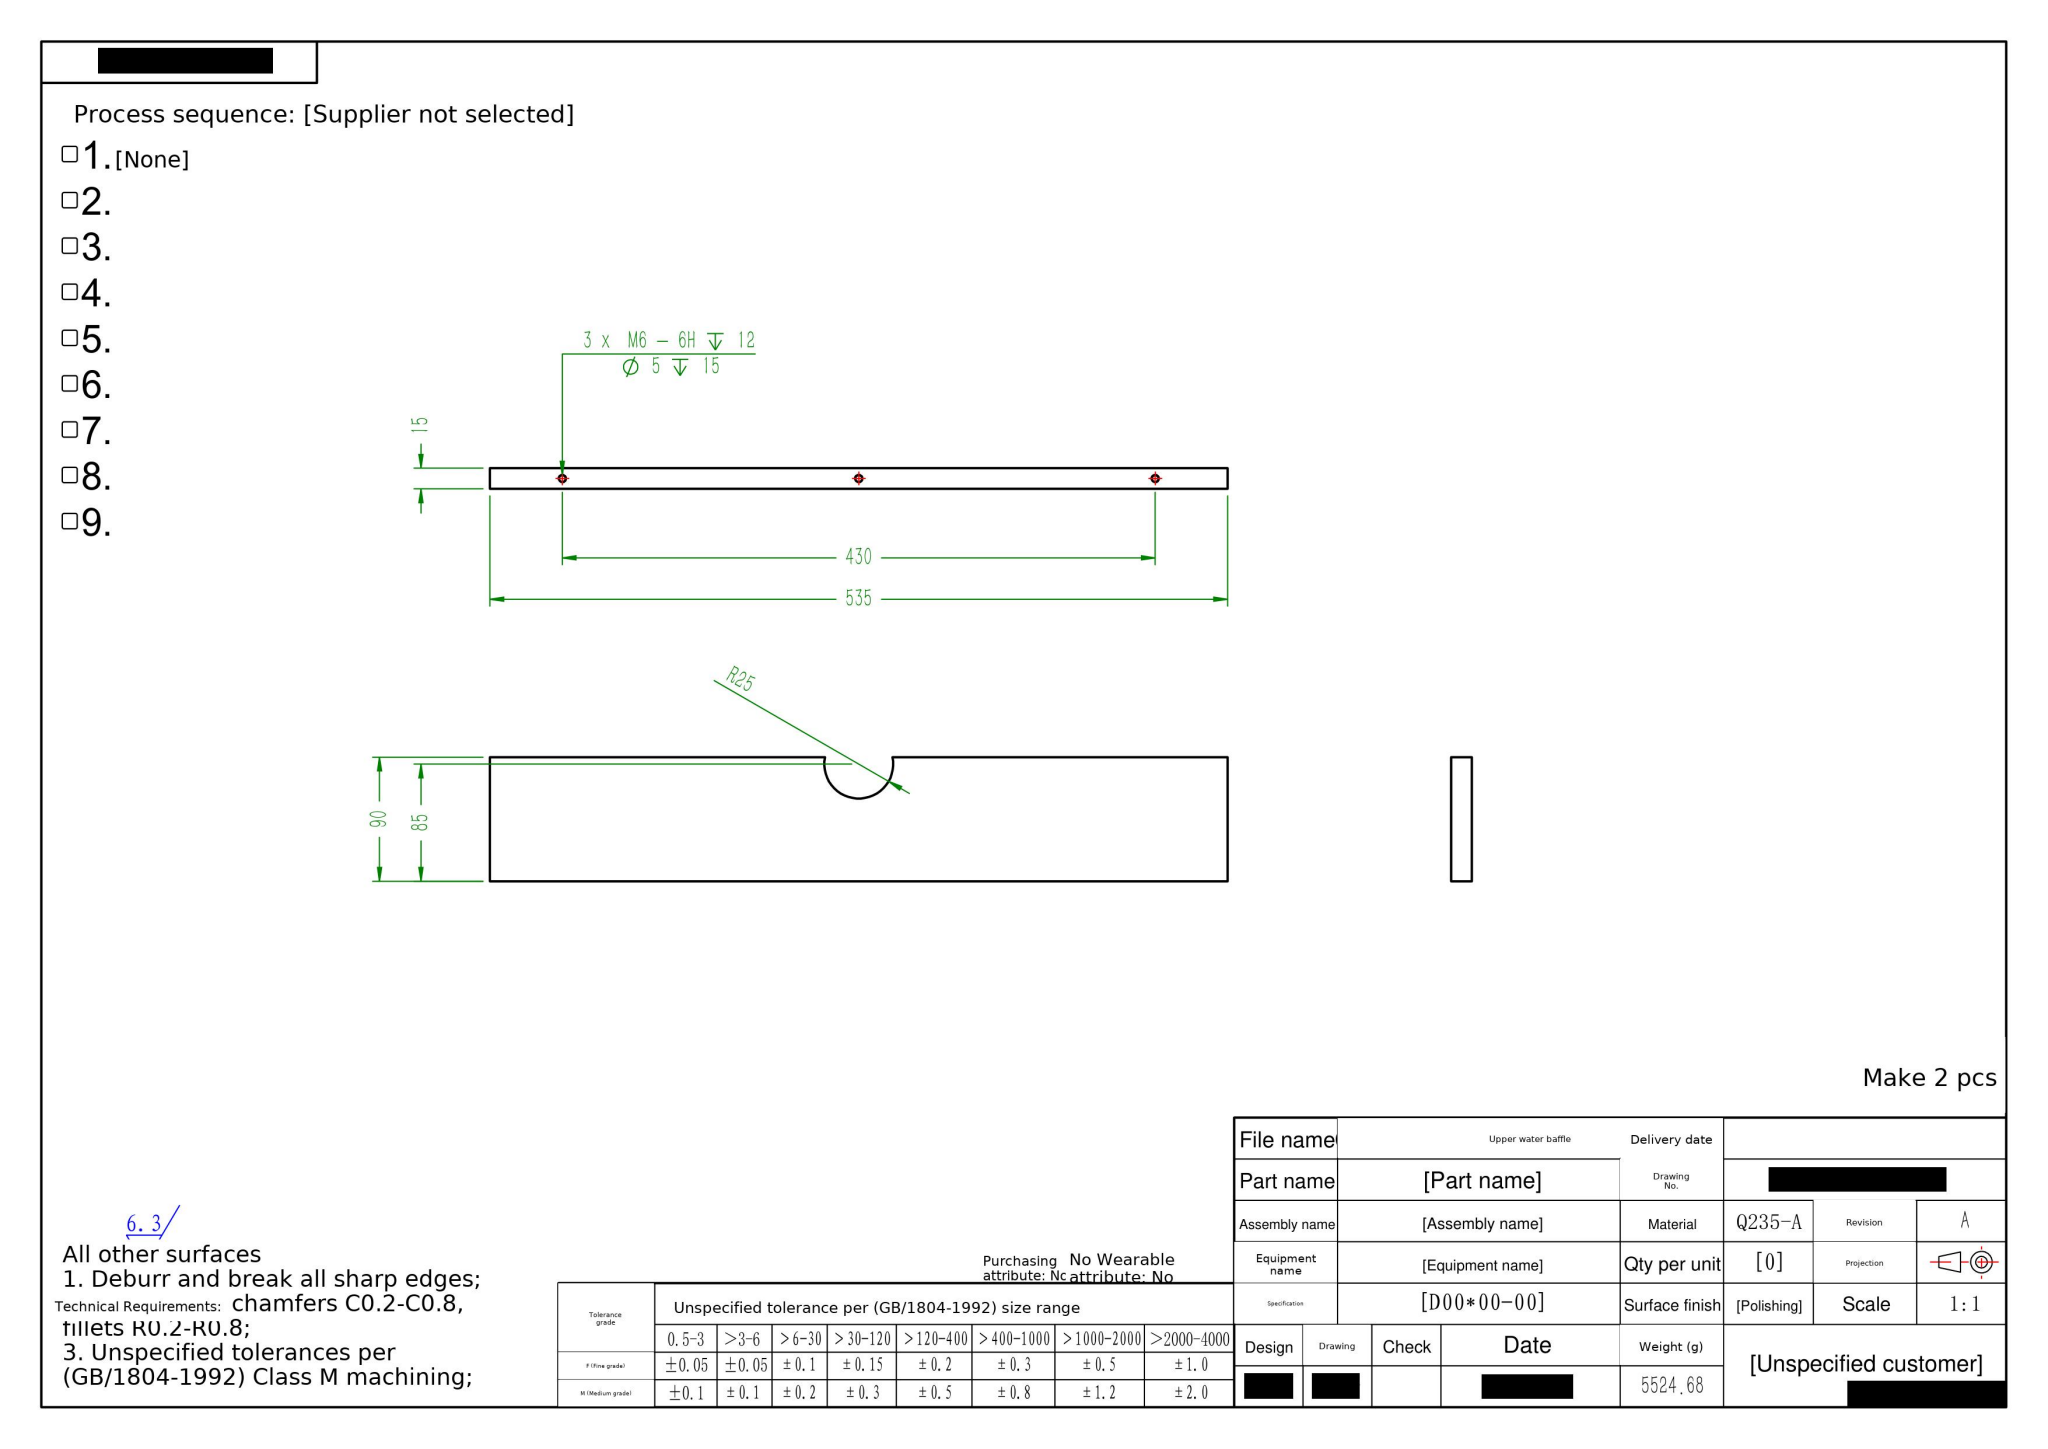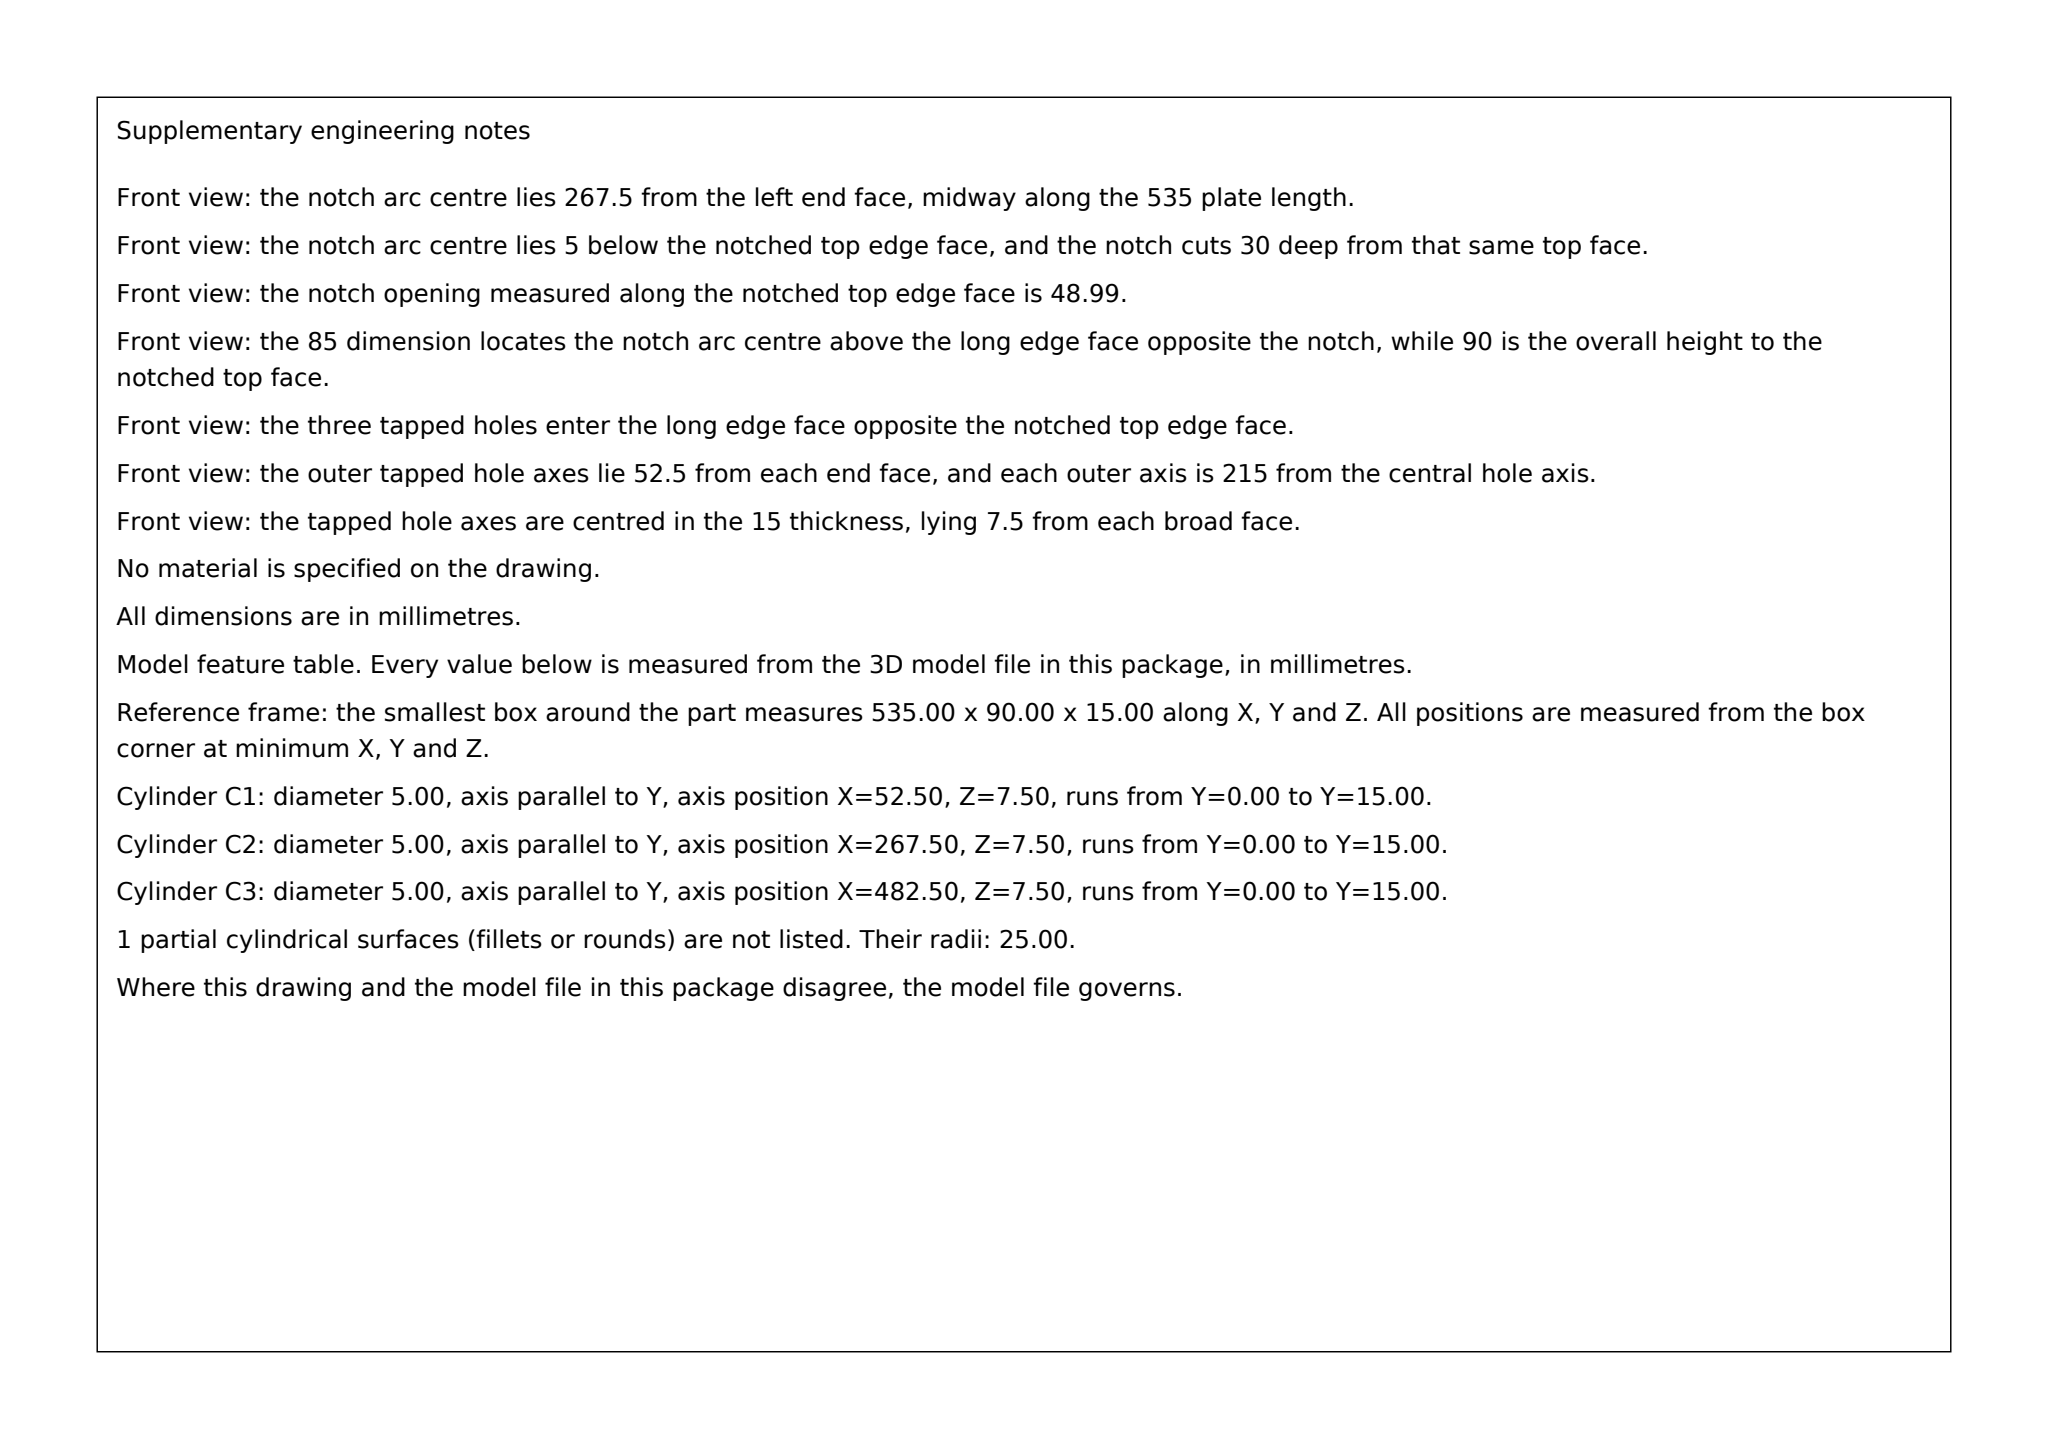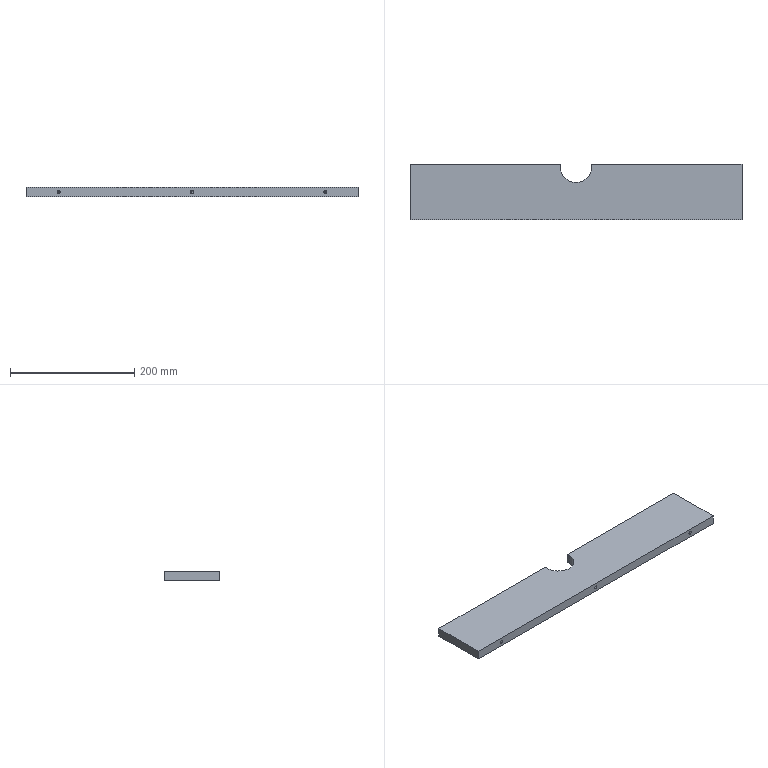Part | SolidWorks | mm | material Q235-A | 1 solid | 22 faces | box 535 x 90 x 15 mm | volume 702886 mm3 | cylinder 9 | plane 7 | cone 6 | commonest cylinder face diameters 5 x6 50 x3
Drawing notes:
2. BREAK SHARP EDGES: CHAMFERS C0.2-C0.8, FILLETS R0.2-R0.8 | from the solid: STEP lists no fillet radii (fillet_radii: []) and no chamfer faces; only sharp-edge prismatic bbox 535x90x15, so note is a general edge-break requirement
build123d program:
from build123d import *

# Parameters (mm, degrees)
SKETCH1_W             = 535
SKETCH1_H             = 15
BOSS_EXTRUDE1_DEPTH   = 90
M6_TAPPED_HOLE1_D     = 5
M6_TAPPED_HOLE1_DEPTH = 15
M6_TAPPED_HOLE1_TIP   = 1.502
SKETCH5_R             = 25
CUT_EXTRUDE2_DEPTH    = 283.633


with BuildPart() as part:
    # Sketch1 → Boss-Extrude1 (new body)
    with BuildSketch(Plane(origin=(0, 0, 0), x_dir=(1, 0, 0), z_dir=(0, 1, 0))):
        Rectangle(SKETCH1_W, SKETCH1_H)
    extrude(amount=BOSS_EXTRUDE1_DEPTH)

    # M6 Tapped Hole1
    with Locations(Plane(origin=(0, 0, 0), x_dir=(-1, 0, 0), z_dir=(0, -1, 0))):
        with Locations((0, 0), (-215, 0), (215, 0)):
            Hole(M6_TAPPED_HOLE1_D / 2, depth=M6_TAPPED_HOLE1_DEPTH)
            with Locations((0, 0, -(M6_TAPPED_HOLE1_DEPTH + M6_TAPPED_HOLE1_TIP / 2))):  # 118° drill point
                Cone(0, M6_TAPPED_HOLE1_D / 2, M6_TAPPED_HOLE1_TIP, mode=Mode.SUBTRACT)

    # Sketch5 → Cut-Extrude2 (cut, through all)
    with BuildSketch(Plane(origin=(0, 0, -7.5), x_dir=(-1, 0, 0), z_dir=(0, 0, -1))):
        with Locations((0, 85)):
            Circle(SKETCH5_R)
    extrude(amount=-CUT_EXTRUDE2_DEPTH, mode=Mode.SUBTRACT)


solid = part.part
STEP:
#1=CARTESIAN_POINT('',(25.,85.,7.5));
#2=VERTEX_POINT('',#1);
#3=CARTESIAN_POINT('',(-25.,85.,7.5));
#4=VERTEX_POINT('',#3);
#5=CARTESIAN_POINT('',(0.,85.,7.5));
#6=DIRECTION('',(0.,0.,-1.));
#7=DIRECTION('',(-1.,0.,0.));
#8=AXIS2_PLACEMENT_3D('',#5,#6,#7);
#9=CIRCLE('',#8,25.);
#10=EDGE_CURVE('',#2,#4,#9,.T.);
#11=ORIENTED_EDGE('',*,*,#10,.F.);
#12=CARTESIAN_POINT('',(25.,85.,-7.5));
#13=VERTEX_POINT('',#12);
#14=CARTESIAN_POINT('',(25.,85.,7.5));
#15=DIRECTION('',(0.,0.,-1.));
#16=VECTOR('',#15,1000.);
#17=LINE('',#14,#16);
#18=EDGE_CURVE('',#2,#13,#17,.T.);
#19=ORIENTED_EDGE('',*,*,#18,.T.);
#20=CARTESIAN_POINT('',(-25.,85.,-7.5));
#21=VERTEX_POINT('',#20);
#22=CARTESIAN_POINT('',(0.,85.,-7.5));
#23=DIRECTION('',(0.,0.,-1.));
#24=DIRECTION('',(-1.,0.,0.));
#25=AXIS2_PLACEMENT_3D('',#22,#23,#24);
#26=CIRCLE('',#25,25.);
#27=EDGE_CURVE('',#13,#21,#26,.T.);
#28=ORIENTED_EDGE('',*,*,#27,.T.);
#29=CARTESIAN_POINT('',(-25.,85.,7.5));
#30=DIRECTION('',(0.,0.,-1.));
#31=VECTOR('',#30,1000.);
#32=LINE('',#29,#31);
#33=EDGE_CURVE('',#4,#21,#32,.T.);
#34=ORIENTED_EDGE('',*,*,#33,.F.);
#35=EDGE_LOOP('',(#11,#19,#28,#34));
#36=FACE_OUTER_BOUND('',#35,.T.);
#37=CARTESIAN_POINT('',(0.,85.,7.5));
#38=DIRECTION('',(0.,0.,-1.));
#39=DIRECTION('',(-1.,0.,0.));
#40=AXIS2_PLACEMENT_3D('',#37,#38,#39);
#41=CYLINDRICAL_SURFACE('',#40,25.);
#42=ADVANCED_FACE('',(#36),#41,.F.);
#43=CARTESIAN_POINT('',(-24.495,90.,7.5));
#44=VERTEX_POINT('',#43);
#45=CARTESIAN_POINT('',(0.,85.,7.5));
#46=DIRECTION('',(0.,0.,-1.));
#47=DIRECTION('',(-1.,0.,0.));
#48=AXIS2_PLACEMENT_3D('',#45,#46,#47);
#49=CIRCLE('',#48,25.);
#50=EDGE_CURVE('',#4,#44,#49,.T.);
#51=ORIENTED_EDGE('',*,*,#50,.F.);
#52=ORIENTED_EDGE('',*,*,#33,.T.);
#53=CARTESIAN_POINT('',(-24.495,90.,-7.5));
#54=VERTEX_POINT('',#53);
#55=CARTESIAN_POINT('',(0.,85.,-7.5));
#56=DIRECTION('',(0.,0.,-1.));
#57=DIRECTION('',(-1.,0.,0.));
#58=AXIS2_PLACEMENT_3D('',#55,#56,#57);
#59=CIRCLE('',#58,25.);
#60=EDGE_CURVE('',#21,#54,#59,.T.);
#61=ORIENTED_EDGE('',*,*,#60,.T.);
#62=CARTESIAN_POINT('',(-24.495,90.,7.5));
#63=DIRECTION('',(0.,0.,-1.));
#64=VECTOR('',#63,1000.);
#65=LINE('',#62,#64);
#66=EDGE_CURVE('',#44,#54,#65,.T.);
#67=ORIENTED_EDGE('',*,*,#66,.F.);
#68=EDGE_LOOP('',(#51,#52,#61,#67));
#69=FACE_OUTER_BOUND('',#68,.T.);
#70=CARTESIAN_POINT('',(0.,85.,7.5));
#71=DIRECTION('',(0.,0.,-1.));
#72=DIRECTION('',(-1.,0.,0.));
#73=AXIS2_PLACEMENT_3D('',#70,#71,#72);
#74=CYLINDRICAL_SURFACE('',#73,25.);
#75=ADVANCED_FACE('',(#69),#74,.F.);
#76=CARTESIAN_POINT('',(0.,15.,2.5));
#77=VERTEX_POINT('',#76);
#78=CARTESIAN_POINT('',(0.,15.,-2.5));
#79=VERTEX_POINT('',#78);
#80=CARTESIAN_POINT('',(0.,15.,0.));
#81=DIRECTION('',(0.,-1.,0.));
#82=DIRECTION('',(0.,0.,-1.));
#83=AXIS2_PLACEMENT_3D('',#80,#81,#82);
#84=CIRCLE('',#83,2.5);
#85=EDGE_CURVE('',#77,#79,#84,.T.);
#86=ORIENTED_EDGE('',*,*,#85,.F.);
#87=CARTESIAN_POINT('',(0.,-0.,2.5));
#88=VERTEX_POINT('',#87);
#89=CARTESIAN_POINT('',(0.,0.,2.5));
#90=DIRECTION('',(0.,-1.,0.));
#91=VECTOR('',#90,1000.);
#92=LINE('',#89,#91);
#93=EDGE_CURVE('',#77,#88,#92,.T.);
#94=ORIENTED_EDGE('',*,*,#93,.T.);
#95=CARTESIAN_POINT('',(0.,-0.,-2.5));
#96=VERTEX_POINT('',#95);
#97=CARTESIAN_POINT('',(0.,-0.,0.));
#98=DIRECTION('',(0.,-1.,0.));
#99=DIRECTION('',(0.,0.,-1.));
#100=AXIS2_PLACEMENT_3D('',#97,#98,#99);
#101=CIRCLE('',#100,2.5);
#102=EDGE_CURVE('',#88,#96,#101,.T.);
#103=ORIENTED_EDGE('',*,*,#102,.T.);
#104=CARTESIAN_POINT('',(0.,0.,-2.5));
#105=DIRECTION('',(0.,-1.,0.));
#106=VECTOR('',#105,1000.);
#107=LINE('',#104,#106);
#108=EDGE_CURVE('',#79,#96,#107,.T.);
#109=ORIENTED_EDGE('',*,*,#108,.F.);
#110=EDGE_LOOP('',(#86,#94,#103,#109));
#111=FACE_OUTER_BOUND('',#110,.T.);
#112=CARTESIAN_POINT('',(0.,0.,0.));
#113=DIRECTION('',(0.,-1.,0.));
#114=DIRECTION('',(0.,0.,-1.));
#115=AXIS2_PLACEMENT_3D('',#112,#113,#114);
#116=CYLINDRICAL_SURFACE('',#115,2.5);
#117=ADVANCED_FACE('',(#111),#116,.F.);
#118=CARTESIAN_POINT('',(-0.,16.502,0.));
#119=VERTEX_POINT('',#118);
#120=CARTESIAN_POINT('',(0.,15.,-2.5));
#121=DIRECTION('',(0.,-0.515,-0.8572));
#122=VECTOR('',#121,1000.);
#123=LINE('',#120,#122);
#124=EDGE_CURVE('',#119,#79,#123,.T.);
#125=ORIENTED_EDGE('',*,*,#124,.F.);
#126=CARTESIAN_POINT('',(0.,15.,2.5));
#127=DIRECTION('',(0.,-0.515,0.8572));
#128=VECTOR('',#127,1000.);
#129=LINE('',#126,#128);
#130=EDGE_CURVE('',#119,#77,#129,.T.);
#131=ORIENTED_EDGE('',*,*,#130,.T.);
#132=ORIENTED_EDGE('',*,*,#85,.T.);
#133=EDGE_LOOP('',(#125,#131,#132));
#134=FACE_OUTER_BOUND('',#133,.T.);
#135=CARTESIAN_POINT('',(0.,15.,0.));
#136=DIRECTION('',(0.,-1.,0.));
#137=DIRECTION('',(0.,0.,-1.));
#138=AXIS2_PLACEMENT_3D('',#135,#136,#137);
#139=CONICAL_SURFACE('',#138,2.5,1.03);
#140=ADVANCED_FACE('',(#134),#139,.F.);
#141=CARTESIAN_POINT('',(215.,15.,2.5));
#142=VERTEX_POINT('',#141);
#143=CARTESIAN_POINT('',(215.,15.,-2.5));
#144=VERTEX_POINT('',#143);
#145=CARTESIAN_POINT('',(215.,15.,0.));
#146=DIRECTION('',(0.,-1.,0.));
#147=DIRECTION('',(0.,0.,-1.));
#148=AXIS2_PLACEMENT_3D('',#145,#146,#147);
#149=CIRCLE('',#148,2.5);
#150=EDGE_CURVE('',#142,#144,#149,.T.);
#151=ORIENTED_EDGE('',*,*,#150,.F.);
#152=CARTESIAN_POINT('',(215.,-0.,2.5));
#153=VERTEX_POINT('',#152);
#154=CARTESIAN_POINT('',(215.,0.,2.5));
#155=DIRECTION('',(0.,-1.,0.));
#156=VECTOR('',#155,1000.);
#157=LINE('',#154,#156);
#158=EDGE_CURVE('',#142,#153,#157,.T.);
#159=ORIENTED_EDGE('',*,*,#158,.T.);
#160=CARTESIAN_POINT('',(215.,-0.,-2.5));
#161=VERTEX_POINT('',#160);
#162=CARTESIAN_POINT('',(215.,-0.,0.));
#163=DIRECTION('',(0.,-1.,0.));
#164=DIRECTION('',(0.,0.,-1.));
#165=AXIS2_PLACEMENT_3D('',#162,#163,#164);
#166=CIRCLE('',#165,2.5);
#167=EDGE_CURVE('',#153,#161,#166,.T.);
#168=ORIENTED_EDGE('',*,*,#167,.T.);
#169=CARTESIAN_POINT('',(215.,0.,-2.5));
#170=DIRECTION('',(0.,-1.,0.));
#171=VECTOR('',#170,1000.);
#172=LINE('',#169,#171);
#173=EDGE_CURVE('',#144,#161,#172,.T.);
#174=ORIENTED_EDGE('',*,*,#173,.F.);
#175=EDGE_LOOP('',(#151,#159,#168,#174));
#176=FACE_OUTER_BOUND('',#175,.T.);
#177=CARTESIAN_POINT('',(215.,0.,0.));
#178=DIRECTION('',(0.,-1.,0.));
#179=DIRECTION('',(0.,0.,-1.));
#180=AXIS2_PLACEMENT_3D('',#177,#178,#179);
#181=CYLINDRICAL_SURFACE('',#180,2.5);
#182=ADVANCED_FACE('',(#176),#181,.F.);
#183=CARTESIAN_POINT('',(215.,16.502,0.));
#184=VERTEX_POINT('',#183);
#185=CARTESIAN_POINT('',(215.,15.,-2.5));
#186=DIRECTION('',(0.,-0.515,-0.8572));
#187=VECTOR('',#186,1000.);
#188=LINE('',#185,#187);
#189=EDGE_CURVE('',#184,#144,#188,.T.);
#190=ORIENTED_EDGE('',*,*,#189,.F.);
#191=CARTESIAN_POINT('',(215.,15.,2.5));
#192=DIRECTION('',(0.,-0.515,0.8572));
#193=VECTOR('',#192,1000.);
#194=LINE('',#191,#193);
#195=EDGE_CURVE('',#184,#142,#194,.T.);
#196=ORIENTED_EDGE('',*,*,#195,.T.);
#197=ORIENTED_EDGE('',*,*,#150,.T.);
#198=EDGE_LOOP('',(#190,#196,#197));
#199=FACE_OUTER_BOUND('',#198,.T.);
#200=CARTESIAN_POINT('',(215.,15.,0.));
#201=DIRECTION('',(0.,-1.,0.));
#202=DIRECTION('',(0.,0.,-1.));
#203=AXIS2_PLACEMENT_3D('',#200,#201,#202);
#204=CONICAL_SURFACE('',#203,2.5,1.03);
#205=ADVANCED_FACE('',(#199),#204,.F.);
#206=CARTESIAN_POINT('',(-215.,15.,2.5));
#207=VERTEX_POINT('',#206);
#208=CARTESIAN_POINT('',(-215.,15.,-2.5));
#209=VERTEX_POINT('',#208);
#210=CARTESIAN_POINT('',(-215.,15.,0.));
#211=DIRECTION('',(0.,-1.,0.));
#212=DIRECTION('',(0.,0.,-1.));
#213=AXIS2_PLACEMENT_3D('',#210,#211,#212);
#214=CIRCLE('',#213,2.5);
#215=EDGE_CURVE('',#207,#209,#214,.T.);
#216=ORIENTED_EDGE('',*,*,#215,.F.);
#217=CARTESIAN_POINT('',(-215.,-0.,2.5));
#218=VERTEX_POINT('',#217);
#219=CARTESIAN_POINT('',(-215.,0.,2.5));
#220=DIRECTION('',(0.,-1.,0.));
#221=VECTOR('',#220,1000.);
#222=LINE('',#219,#221);
#223=EDGE_CURVE('',#207,#218,#222,.T.);
#224=ORIENTED_EDGE('',*,*,#223,.T.);
#225=CARTESIAN_POINT('',(-215.,-0.,-2.5));
#226=VERTEX_POINT('',#225);
#227=CARTESIAN_POINT('',(-215.,-0.,0.));
#228=DIRECTION('',(0.,-1.,0.));
#229=DIRECTION('',(0.,0.,-1.));
#230=AXIS2_PLACEMENT_3D('',#227,#228,#229);
#231=CIRCLE('',#230,2.5);
#232=EDGE_CURVE('',#218,#226,#231,.T.);
#233=ORIENTED_EDGE('',*,*,#232,.T.);
#234=CARTESIAN_POINT('',(-215.,0.,-2.5));
#235=DIRECTION('',(0.,-1.,0.));
#236=VECTOR('',#235,1000.);
#237=LINE('',#234,#236);
#238=EDGE_CURVE('',#209,#226,#237,.T.);
#239=ORIENTED_EDGE('',*,*,#238,.F.);
#240=EDGE_LOOP('',(#216,#224,#233,#239));
#241=FACE_OUTER_BOUND('',#240,.T.);
#242=CARTESIAN_POINT('',(-215.,0.,0.));
#243=DIRECTION('',(0.,-1.,0.));
#244=DIRECTION('',(0.,0.,-1.));
#245=AXIS2_PLACEMENT_3D('',#242,#243,#244);
#246=CYLINDRICAL_SURFACE('',#245,2.5);
#247=ADVANCED_FACE('',(#241),#246,.F.);
#248=CARTESIAN_POINT('',(-215.,16.502,0.));
#249=VERTEX_POINT('',#248);
#250=CARTESIAN_POINT('',(-215.,15.,-2.5));
#251=DIRECTION('',(0.,-0.515,-0.8572));
#252=VECTOR('',#251,1000.);
#253=LINE('',#250,#252);
#254=EDGE_CURVE('',#249,#209,#253,.T.);
#255=ORIENTED_EDGE('',*,*,#254,.F.);
#256=CARTESIAN_POINT('',(-215.,15.,2.5));
#257=DIRECTION('',(0.,-0.515,0.8572));
#258=VECTOR('',#257,1000.);
#259=LINE('',#256,#258);
#260=EDGE_CURVE('',#249,#207,#259,.T.);
#261=ORIENTED_EDGE('',*,*,#260,.T.);
#262=ORIENTED_EDGE('',*,*,#215,.T.);
#263=EDGE_LOOP('',(#255,#261,#262));
#264=FACE_OUTER_BOUND('',#263,.T.);
#265=CARTESIAN_POINT('',(-215.,15.,0.));
#266=DIRECTION('',(0.,-1.,0.));
#267=DIRECTION('',(0.,0.,-1.));
#268=AXIS2_PLACEMENT_3D('',#265,#266,#267);
#269=CONICAL_SURFACE('',#268,2.5,1.03);
#270=ADVANCED_FACE('',(#264),#269,.F.);
#271=CARTESIAN_POINT('',(-267.5,90.,7.5));
#272=VERTEX_POINT('',#271);
#273=CARTESIAN_POINT('',(267.5,90.,7.5));
#274=DIRECTION('',(1.,0.,0.));
#275=VECTOR('',#274,1000.);
#276=LINE('',#273,#275);
#277=EDGE_CURVE('',#272,#44,#276,.T.);
#278=ORIENTED_EDGE('',*,*,#277,.T.);
#279=ORIENTED_EDGE('',*,*,#66,.T.);
#280=CARTESIAN_POINT('',(-267.5,90.,-7.5));
#281=VERTEX_POINT('',#280);
#282=CARTESIAN_POINT('',(267.5,90.,-7.5));
#283=DIRECTION('',(-1.,0.,0.));
#284=VECTOR('',#283,1000.);
#285=LINE('',#282,#284);
#286=EDGE_CURVE('',#54,#281,#285,.T.);
#287=ORIENTED_EDGE('',*,*,#286,.T.);
#288=CARTESIAN_POINT('',(-267.5,90.,-7.5));
#289=DIRECTION('',(0.,0.,1.));
#290=VECTOR('',#289,1000.);
#291=LINE('',#288,#290);
#292=EDGE_CURVE('',#281,#272,#291,.T.);
#293=ORIENTED_EDGE('',*,*,#292,.T.);
#294=EDGE_LOOP('',(#278,#279,#287,#293));
#295=FACE_OUTER_BOUND('',#294,.T.);
#296=CARTESIAN_POINT('',(0.,90.,0.));
#297=DIRECTION('',(0.,-1.,0.));
#298=DIRECTION('',(0.,0.,-1.));
#299=AXIS2_PLACEMENT_3D('',#296,#297,#298);
#300=PLANE('',#299);
#301=ADVANCED_FACE('',(#295),#300,.F.);
#302=CARTESIAN_POINT('',(-267.5,0.,-7.5));
#303=VERTEX_POINT('',#302);
#304=CARTESIAN_POINT('',(-267.5,0.,7.5));
#305=VERTEX_POINT('',#304);
#306=CARTESIAN_POINT('',(-267.5,0.,-7.5));
#307=DIRECTION('',(0.,0.,1.));
#308=VECTOR('',#307,1000.);
#309=LINE('',#306,#308);
#310=EDGE_CURVE('',#303,#305,#309,.T.);
#311=ORIENTED_EDGE('',*,*,#310,.T.);
#312=CARTESIAN_POINT('',(-267.5,90.,7.5));
#313=DIRECTION('',(0.,-1.,0.));
#314=VECTOR('',#313,1000.);
#315=LINE('',#312,#314);
#316=EDGE_CURVE('',#272,#305,#315,.T.);
#317=ORIENTED_EDGE('',*,*,#316,.F.);
#318=ORIENTED_EDGE('',*,*,#292,.F.);
#319=CARTESIAN_POINT('',(-267.5,90.,-7.5));
#320=DIRECTION('',(0.,-1.,0.));
#321=VECTOR('',#320,1000.);
#322=LINE('',#319,#321);
#323=EDGE_CURVE('',#281,#303,#322,.T.);
#324=ORIENTED_EDGE('',*,*,#323,.T.);
#325=EDGE_LOOP('',(#311,#317,#318,#324));
#326=FACE_OUTER_BOUND('',#325,.T.);
#327=CARTESIAN_POINT('',(-267.5,90.,-7.5));
#328=DIRECTION('',(1.,0.,0.));
#329=DIRECTION('',(0.,0.,-1.));
#330=AXIS2_PLACEMENT_3D('',#327,#328,#329);
#331=PLANE('',#330);
#332=ADVANCED_FACE('',(#326),#331,.F.);
#333=CARTESIAN_POINT('',(24.495,90.,7.5));
#334=VERTEX_POINT('',#333);
#335=CARTESIAN_POINT('',(267.5,90.,7.5));
#336=VERTEX_POINT('',#335);
#337=CARTESIAN_POINT('',(267.5,90.,7.5));
#338=DIRECTION('',(1.,0.,0.));
#339=VECTOR('',#338,1000.);
#340=LINE('',#337,#339);
#341=EDGE_CURVE('',#334,#336,#340,.T.);
#342=ORIENTED_EDGE('',*,*,#341,.F.);
#343=CARTESIAN_POINT('',(0.,85.,7.5));
#344=DIRECTION('',(0.,0.,-1.));
#345=DIRECTION('',(-1.,0.,0.));
#346=AXIS2_PLACEMENT_3D('',#343,#344,#345);
#347=CIRCLE('',#346,25.);
#348=EDGE_CURVE('',#334,#2,#347,.T.);
#349=ORIENTED_EDGE('',*,*,#348,.T.);
#350=ORIENTED_EDGE('',*,*,#10,.T.);
#351=ORIENTED_EDGE('',*,*,#50,.T.);
#352=ORIENTED_EDGE('',*,*,#277,.F.);
#353=ORIENTED_EDGE('',*,*,#316,.T.);
#354=CARTESIAN_POINT('',(267.5,0.,7.5));
#355=VERTEX_POINT('',#354);
#356=CARTESIAN_POINT('',(267.5,0.,7.5));
#357=DIRECTION('',(1.,0.,0.));
#358=VECTOR('',#357,1000.);
#359=LINE('',#356,#358);
#360=EDGE_CURVE('',#305,#355,#359,.T.);
#361=ORIENTED_EDGE('',*,*,#360,.T.);
#362=CARTESIAN_POINT('',(267.5,90.,7.5));
#363=DIRECTION('',(0.,-1.,0.));
#364=VECTOR('',#363,1000.);
#365=LINE('',#362,#364);
#366=EDGE_CURVE('',#336,#355,#365,.T.);
#367=ORIENTED_EDGE('',*,*,#366,.F.);
#368=EDGE_LOOP('',(#342,#349,#350,#351,#352,#353,#361,#367));
#369=FACE_OUTER_BOUND('',#368,.T.);
#370=CARTESIAN_POINT('',(267.5,90.,7.5));
#371=DIRECTION('',(0.,0.,-1.));
#372=DIRECTION('',(-1.,0.,0.));
#373=AXIS2_PLACEMENT_3D('',#370,#371,#372);
#374=PLANE('',#373);
#375=ADVANCED_FACE('',(#369),#374,.F.);
#376=CARTESIAN_POINT('',(267.5,0.,-7.5));
#377=VERTEX_POINT('',#376);
#378=CARTESIAN_POINT('',(267.5,0.,-7.5));
#379=DIRECTION('',(0.,0.,-1.));
#380=VECTOR('',#379,1000.);
#381=LINE('',#378,#380);
#382=EDGE_CURVE('',#355,#377,#381,.T.);
#383=ORIENTED_EDGE('',*,*,#382,.T.);
#384=CARTESIAN_POINT('',(267.5,90.,-7.5));
#385=VERTEX_POINT('',#384);
#386=CARTESIAN_POINT('',(267.5,90.,-7.5));
#387=DIRECTION('',(0.,-1.,0.));
#388=VECTOR('',#387,1000.);
#389=LINE('',#386,#388);
#390=EDGE_CURVE('',#385,#377,#389,.T.);
#391=ORIENTED_EDGE('',*,*,#390,.F.);
#392=CARTESIAN_POINT('',(267.5,90.,-7.5));
#393=DIRECTION('',(0.,0.,-1.));
#394=VECTOR('',#393,1000.);
#395=LINE('',#392,#394);
#396=EDGE_CURVE('',#336,#385,#395,.T.);
#397=ORIENTED_EDGE('',*,*,#396,.F.);
#398=ORIENTED_EDGE('',*,*,#366,.T.);
#399=EDGE_LOOP('',(#383,#391,#397,#398));
#400=FACE_OUTER_BOUND('',#399,.T.);
#401=CARTESIAN_POINT('',(267.5,90.,-7.5));
#402=DIRECTION('',(-1.,0.,0.));
#403=DIRECTION('',(0.,0.,1.));
#404=AXIS2_PLACEMENT_3D('',#401,#402,#403);
#405=PLANE('',#404);
#406=ADVANCED_FACE('',(#400),#405,.F.);
#407=ORIENTED_EDGE('',*,*,#286,.F.);
#408=ORIENTED_EDGE('',*,*,#60,.F.);
#409=ORIENTED_EDGE('',*,*,#27,.F.);
#410=CARTESIAN_POINT('',(24.495,90.,-7.5));
#411=VERTEX_POINT('',#410);
#412=CARTESIAN_POINT('',(0.,85.,-7.5));
#413=DIRECTION('',(0.,0.,-1.));
#414=DIRECTION('',(-1.,0.,0.));
#415=AXIS2_PLACEMENT_3D('',#412,#413,#414);
#416=CIRCLE('',#415,25.);
#417=EDGE_CURVE('',#411,#13,#416,.T.);
#418=ORIENTED_EDGE('',*,*,#417,.F.);
#419=CARTESIAN_POINT('',(267.5,90.,-7.5));
#420=DIRECTION('',(-1.,0.,0.));
#421=VECTOR('',#420,1000.);
#422=LINE('',#419,#421);
#423=EDGE_CURVE('',#385,#411,#422,.T.);
#424=ORIENTED_EDGE('',*,*,#423,.F.);
#425=ORIENTED_EDGE('',*,*,#390,.T.);
#426=CARTESIAN_POINT('',(267.5,0.,-7.5));
#427=DIRECTION('',(-1.,0.,0.));
#428=VECTOR('',#427,1000.);
#429=LINE('',#426,#428);
#430=EDGE_CURVE('',#377,#303,#429,.T.);
#431=ORIENTED_EDGE('',*,*,#430,.T.);
#432=ORIENTED_EDGE('',*,*,#323,.F.);
#433=EDGE_LOOP('',(#407,#408,#409,#418,#424,#425,#431,#432));
#434=FACE_OUTER_BOUND('',#433,.T.);
#435=CARTESIAN_POINT('',(267.5,90.,-7.5));
#436=DIRECTION('',(0.,0.,1.));
#437=DIRECTION('',(1.,0.,0.));
#438=AXIS2_PLACEMENT_3D('',#435,#436,#437);
#439=PLANE('',#438);
#440=ADVANCED_FACE('',(#434),#439,.F.);
#441=ORIENTED_EDGE('',*,*,#423,.T.);
#442=CARTESIAN_POINT('',(24.495,90.,7.5));
#443=DIRECTION('',(0.,0.,1.));
#444=VECTOR('',#443,1000.);
#445=LINE('',#442,#444);
#446=EDGE_CURVE('',#411,#334,#445,.T.);
#447=ORIENTED_EDGE('',*,*,#446,.T.);
#448=ORIENTED_EDGE('',*,*,#341,.T.);
#449=ORIENTED_EDGE('',*,*,#396,.T.);
#450=EDGE_LOOP('',(#441,#447,#448,#449));
#451=FACE_OUTER_BOUND('',#450,.T.);
#452=CARTESIAN_POINT('',(0.,90.,0.));
#453=DIRECTION('',(0.,-1.,0.));
#454=DIRECTION('',(0.,0.,-1.));
#455=AXIS2_PLACEMENT_3D('',#452,#453,#454);
#456=PLANE('',#455);
#457=ADVANCED_FACE('',(#451),#456,.F.);
#458=CARTESIAN_POINT('',(0.,-0.,0.));
#459=DIRECTION('',(0.,-1.,0.));
#460=DIRECTION('',(0.,0.,-1.));
#461=AXIS2_PLACEMENT_3D('',#458,#459,#460);
#462=CIRCLE('',#461,2.5);
#463=EDGE_CURVE('',#96,#88,#462,.T.);
#464=ORIENTED_EDGE('',*,*,#463,.F.);
#465=ORIENTED_EDGE('',*,*,#102,.F.);
#466=EDGE_LOOP('',(#464,#465));
#467=FACE_BOUND('',#466,.T.);
#468=CARTESIAN_POINT('',(215.,-0.,0.));
#469=DIRECTION('',(0.,-1.,0.));
#470=DIRECTION('',(0.,0.,-1.));
#471=AXIS2_PLACEMENT_3D('',#468,#469,#470);
#472=CIRCLE('',#471,2.5);
#473=EDGE_CURVE('',#161,#153,#472,.T.);
#474=ORIENTED_EDGE('',*,*,#473,.F.);
#475=ORIENTED_EDGE('',*,*,#167,.F.);
#476=EDGE_LOOP('',(#474,#475));
#477=FACE_BOUND('',#476,.T.);
#478=CARTESIAN_POINT('',(-215.,-0.,0.));
#479=DIRECTION('',(0.,-1.,0.));
#480=DIRECTION('',(0.,0.,-1.));
#481=AXIS2_PLACEMENT_3D('',#478,#479,#480);
#482=CIRCLE('',#481,2.5);
#483=EDGE_CURVE('',#226,#218,#482,.T.);
#484=ORIENTED_EDGE('',*,*,#483,.F.);
#485=ORIENTED_EDGE('',*,*,#232,.F.);
#486=EDGE_LOOP('',(#484,#485));
#487=FACE_BOUND('',#486,.T.);
#488=ORIENTED_EDGE('',*,*,#310,.F.);
#489=ORIENTED_EDGE('',*,*,#430,.F.);
#490=ORIENTED_EDGE('',*,*,#382,.F.);
#491=ORIENTED_EDGE('',*,*,#360,.F.);
#492=EDGE_LOOP('',(#488,#489,#490,#491));
#493=FACE_OUTER_BOUND('',#492,.T.);
#494=CARTESIAN_POINT('',(0.,0.,0.));
#495=DIRECTION('',(0.,-1.,0.));
#496=DIRECTION('',(0.,0.,-1.));
#497=AXIS2_PLACEMENT_3D('',#494,#495,#496);
#498=PLANE('',#497);
#499=ADVANCED_FACE('',(#467,#477,#487,#493),#498,.T.);
#500=ORIENTED_EDGE('',*,*,#260,.F.);
#501=ORIENTED_EDGE('',*,*,#254,.T.);
#502=CARTESIAN_POINT('',(-215.,15.,0.));
#503=DIRECTION('',(0.,-1.,0.));
#504=DIRECTION('',(0.,0.,-1.));
#505=AXIS2_PLACEMENT_3D('',#502,#503,#504);
#506=CIRCLE('',#505,2.5);
#507=EDGE_CURVE('',#209,#207,#506,.T.);
#508=ORIENTED_EDGE('',*,*,#507,.T.);
#509=EDGE_LOOP('',(#500,#501,#508));
#510=FACE_OUTER_BOUND('',#509,.T.);
#511=CARTESIAN_POINT('',(-215.,15.,0.));
#512=DIRECTION('',(0.,-1.,0.));
#513=DIRECTION('',(0.,0.,-1.));
#514=AXIS2_PLACEMENT_3D('',#511,#512,#513);
#515=CONICAL_SURFACE('',#514,2.5,1.03);
#516=ADVANCED_FACE('',(#510),#515,.F.);
#517=ORIENTED_EDGE('',*,*,#223,.F.);
#518=ORIENTED_EDGE('',*,*,#507,.F.);
#519=ORIENTED_EDGE('',*,*,#238,.T.);
#520=ORIENTED_EDGE('',*,*,#483,.T.);
#521=EDGE_LOOP('',(#517,#518,#519,#520));
#522=FACE_OUTER_BOUND('',#521,.T.);
#523=CARTESIAN_POINT('',(-215.,0.,0.));
#524=DIRECTION('',(0.,-1.,0.));
#525=DIRECTION('',(0.,0.,-1.));
#526=AXIS2_PLACEMENT_3D('',#523,#524,#525);
#527=CYLINDRICAL_SURFACE('',#526,2.5);
#528=ADVANCED_FACE('',(#522),#527,.F.);
#529=ORIENTED_EDGE('',*,*,#195,.F.);
#530=ORIENTED_EDGE('',*,*,#189,.T.);
#531=CARTESIAN_POINT('',(215.,15.,0.));
#532=DIRECTION('',(0.,-1.,0.));
#533=DIRECTION('',(0.,0.,-1.));
#534=AXIS2_PLACEMENT_3D('',#531,#532,#533);
#535=CIRCLE('',#534,2.5);
#536=EDGE_CURVE('',#144,#142,#535,.T.);
#537=ORIENTED_EDGE('',*,*,#536,.T.);
#538=EDGE_LOOP('',(#529,#530,#537));
#539=FACE_OUTER_BOUND('',#538,.T.);
#540=CARTESIAN_POINT('',(215.,15.,0.));
#541=DIRECTION('',(0.,-1.,0.));
#542=DIRECTION('',(0.,0.,-1.));
#543=AXIS2_PLACEMENT_3D('',#540,#541,#542);
#544=CONICAL_SURFACE('',#543,2.5,1.03);
#545=ADVANCED_FACE('',(#539),#544,.F.);
#546=ORIENTED_EDGE('',*,*,#158,.F.);
#547=ORIENTED_EDGE('',*,*,#536,.F.);
#548=ORIENTED_EDGE('',*,*,#173,.T.);
#549=ORIENTED_EDGE('',*,*,#473,.T.);
#550=EDGE_LOOP('',(#546,#547,#548,#549));
#551=FACE_OUTER_BOUND('',#550,.T.);
#552=CARTESIAN_POINT('',(215.,0.,0.));
#553=DIRECTION('',(0.,-1.,0.));
#554=DIRECTION('',(0.,0.,-1.));
#555=AXIS2_PLACEMENT_3D('',#552,#553,#554);
#556=CYLINDRICAL_SURFACE('',#555,2.5);
#557=ADVANCED_FACE('',(#551),#556,.F.);
#558=ORIENTED_EDGE('',*,*,#130,.F.);
#559=ORIENTED_EDGE('',*,*,#124,.T.);
#560=CARTESIAN_POINT('',(0.,15.,0.));
#561=DIRECTION('',(0.,-1.,0.));
#562=DIRECTION('',(0.,0.,-1.));
#563=AXIS2_PLACEMENT_3D('',#560,#561,#562);
#564=CIRCLE('',#563,2.5);
#565=EDGE_CURVE('',#79,#77,#564,.T.);
#566=ORIENTED_EDGE('',*,*,#565,.T.);
#567=EDGE_LOOP('',(#558,#559,#566));
#568=FACE_OUTER_BOUND('',#567,.T.);
#569=CARTESIAN_POINT('',(0.,15.,0.));
#570=DIRECTION('',(0.,-1.,0.));
#571=DIRECTION('',(0.,0.,-1.));
#572=AXIS2_PLACEMENT_3D('',#569,#570,#571);
#573=CONICAL_SURFACE('',#572,2.5,1.03);
#574=ADVANCED_FACE('',(#568),#573,.F.);
#575=ORIENTED_EDGE('',*,*,#93,.F.);
#576=ORIENTED_EDGE('',*,*,#565,.F.);
#577=ORIENTED_EDGE('',*,*,#108,.T.);
#578=ORIENTED_EDGE('',*,*,#463,.T.);
#579=EDGE_LOOP('',(#575,#576,#577,#578));
#580=FACE_OUTER_BOUND('',#579,.T.);
#581=CARTESIAN_POINT('',(0.,0.,0.));
#582=DIRECTION('',(0.,-1.,0.));
#583=DIRECTION('',(0.,0.,-1.));
#584=AXIS2_PLACEMENT_3D('',#581,#582,#583);
#585=CYLINDRICAL_SURFACE('',#584,2.5);
#586=ADVANCED_FACE('',(#580),#585,.F.);
#587=ORIENTED_EDGE('',*,*,#18,.F.);
#588=ORIENTED_EDGE('',*,*,#348,.F.);
#589=ORIENTED_EDGE('',*,*,#446,.F.);
#590=ORIENTED_EDGE('',*,*,#417,.T.);
#591=EDGE_LOOP('',(#587,#588,#589,#590));
#592=FACE_OUTER_BOUND('',#591,.T.);
#593=CARTESIAN_POINT('',(0.,85.,7.5));
#594=DIRECTION('',(0.,0.,-1.));
#595=DIRECTION('',(-1.,0.,0.));
#596=AXIS2_PLACEMENT_3D('',#593,#594,#595);
#597=CYLINDRICAL_SURFACE('',#596,25.);
#598=ADVANCED_FACE('',(#592),#597,.F.);
#599=CLOSED_SHELL('',(#42,#75,#117,#140,#182,#205,#247,#270,#301,#332,#375,#406,#440,#457,#499,#516,#528,#545,#557,#574,#586,#598));
#600=MANIFOLD_SOLID_BREP('',#599);
#601=CARTESIAN_POINT('',(0.,0.,0.));
#602=DIRECTION('',(0.,0.,1.));
#603=DIRECTION('',(1.,0.,0.));
#604=AXIS2_PLACEMENT_3D('',#601,#602,#603);
#605=(LENGTH_UNIT()NAMED_UNIT(*)SI_UNIT(.MILLI.,.METRE.));
#606=UNCERTAINTY_MEASURE_WITH_UNIT(LENGTH_MEASURE(0.00001),#605,'','');
#607=(NAMED_UNIT(*)PLANE_ANGLE_UNIT()SI_UNIT($,.RADIAN.));
#608=(NAMED_UNIT(*)SI_UNIT($,.STERADIAN.)SOLID_ANGLE_UNIT());
#609=(GEOMETRIC_REPRESENTATION_CONTEXT(3)GLOBAL_UNCERTAINTY_ASSIGNED_CONTEXT((#606))GLOBAL_UNIT_ASSIGNED_CONTEXT((#605,#607,#608))REPRESENTATION_CONTEXT('',''));
#610=ADVANCED_BREP_SHAPE_REPRESENTATION('',(#600,#604),#609);